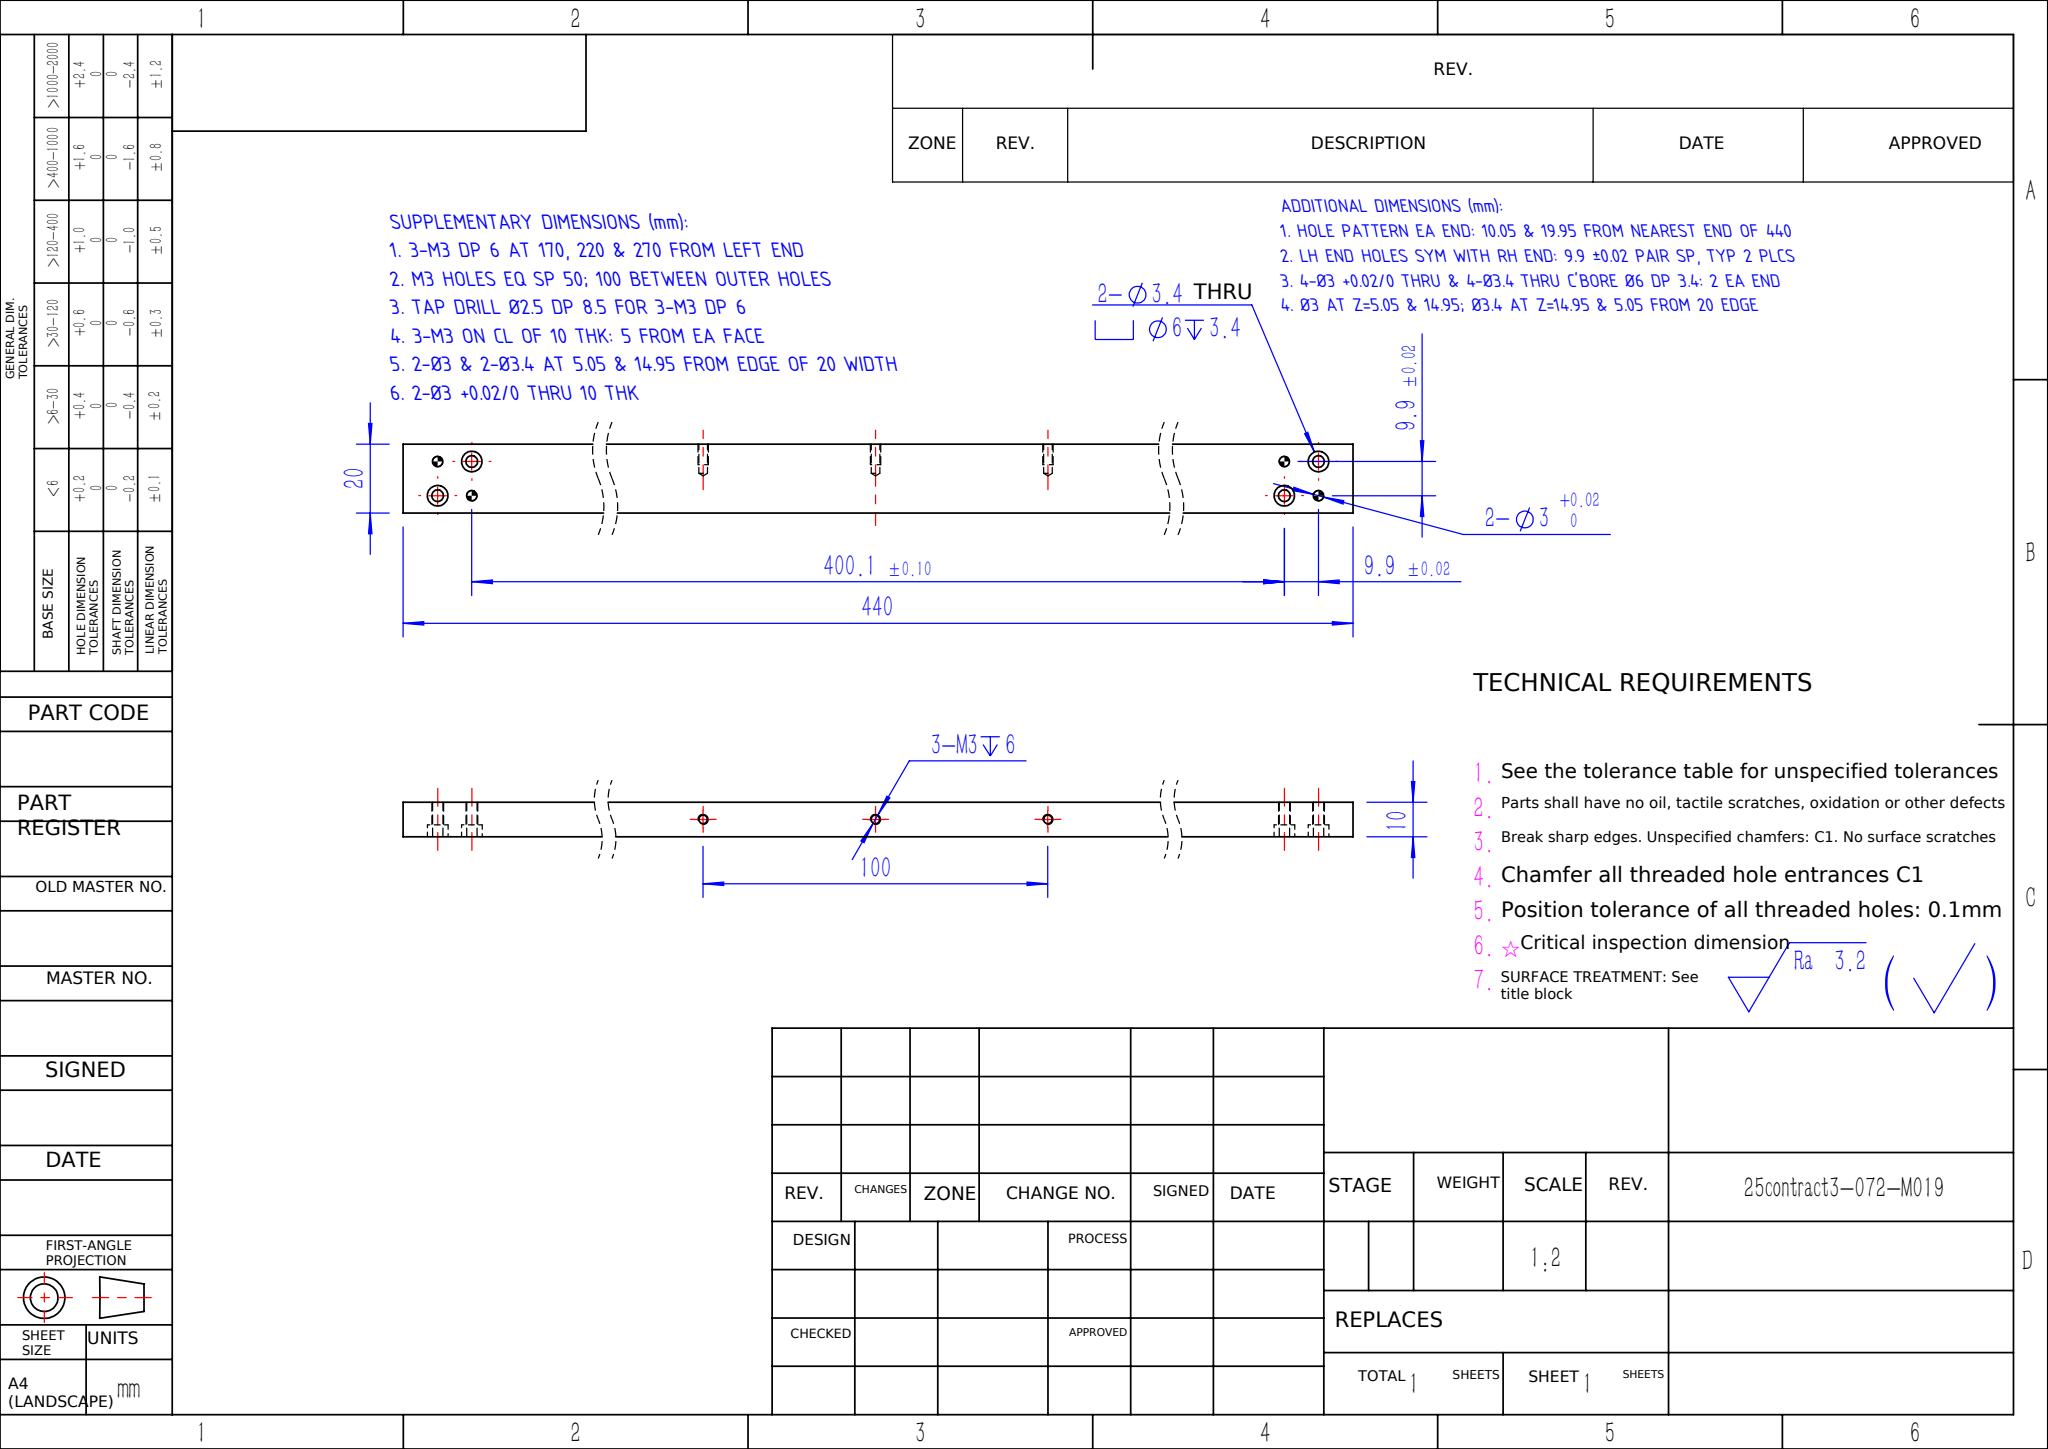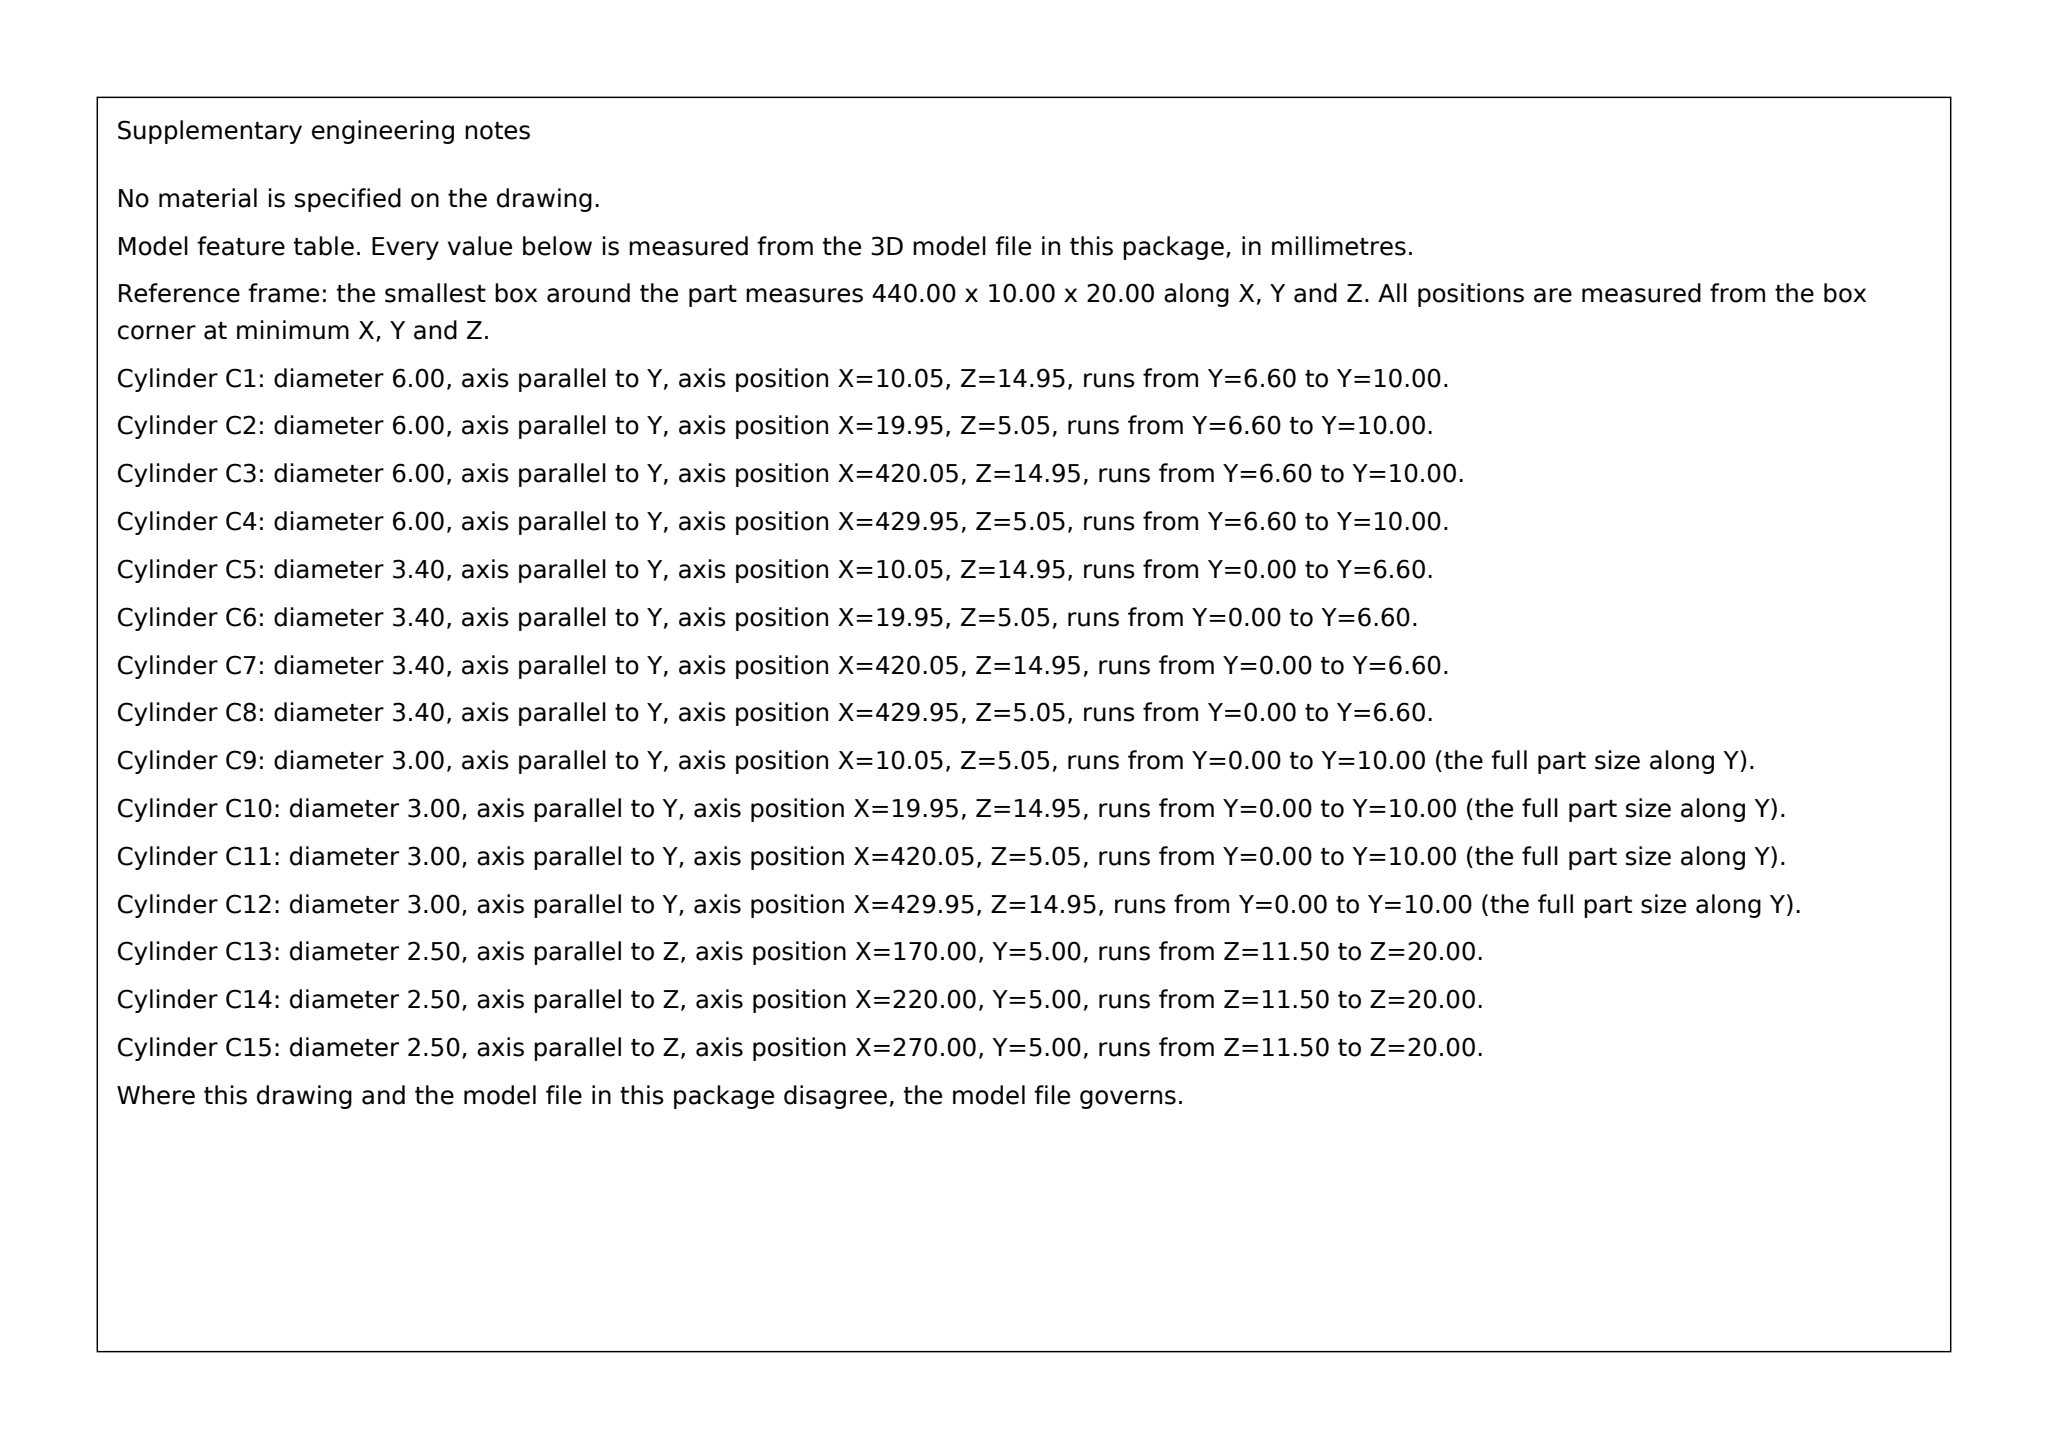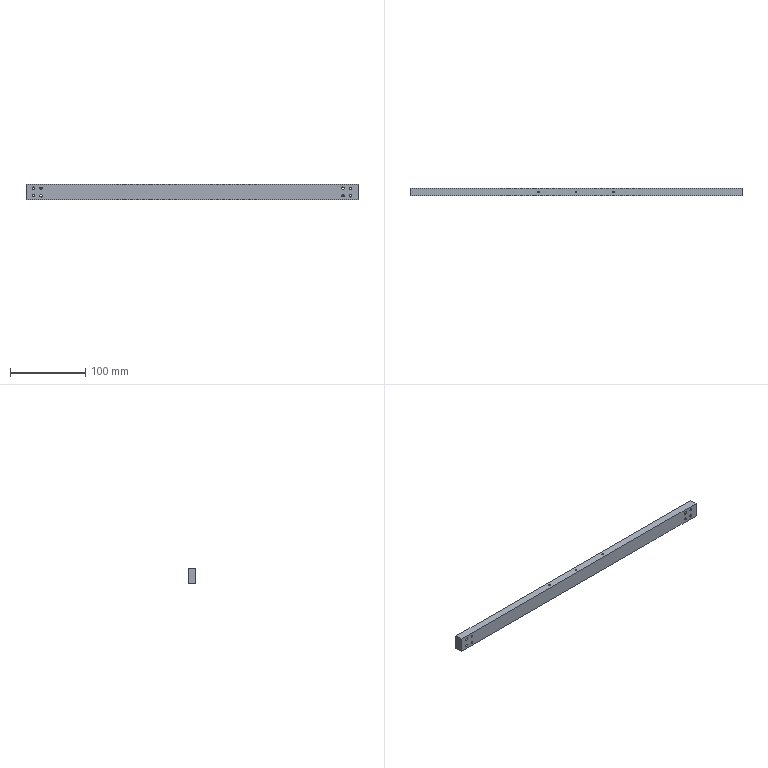Part | SolidWorks | mm | 1 solid | 46 faces | box 440 x 10 x 20 mm | volume 86964 mm3 | cylinder 30 | plane 10 | cone 6 | commonest cylinder face diameters 3 x8 6 x8 3.4 x8 2.5 x6
build123d program:
from build123d import *

# Parameters (mm, degrees)
SKETCH7_W                                         = 440
SKETCH7_H                                         = 20
BOSS_EXTRUDE1_DEPTH                               = 10
HOLE_SIZE_ACCORDING_TO_HEXAGON_SOCKET_D           = 3.4
HOLE_SIZE_ACCORDING_TO_HEXAGON_SOCKET_CBORE_D     = 6
HOLE_SIZE_ACCORDING_TO_HEXAGON_SOCKET_CBORE_DEPTH = 3.4
SIZE_MM_DOWEL_PIN_HOLE1_D                         = 3
M3_TAPPED_HOLE1_D                                 = 2.5
M3_TAPPED_HOLE1_DEPTH                             = 8.5
M3_TAPPED_HOLE1_TIP                               = 0.7511
HOLE_SIZE_ACCORDING_TO_HEXAGON_SO_2_D             = 3.4
HOLE_SIZE_ACCORDING_TO_HEXAGON_SO_2_CBORE_D       = 6
HOLE_SIZE_ACCORDING_TO_HEXAGON_SO_2_CBORE_DEPTH   = 3.4
SIZE_MM_DOWEL_PIN_HOLE2_D                         = 3


with BuildPart() as part:
    # Sketch7 → Boss-Extrude1 (new body)
    with BuildSketch(Plane(origin=(0, 0, 0), x_dir=(1, 0, 0), z_dir=(0, 1, 0))):
        Rectangle(SKETCH7_W, SKETCH7_H)
    extrude(amount=BOSS_EXTRUDE1_DEPTH)

    # Hole Size _ according to_ Hexagon Socket (through all)
    with Locations(Plane(origin=(0, 10, 0), x_dir=(1, 0, 0), z_dir=(0, 1, 0))):
        with Locations((-200.05, 4.95), (-209.95, -4.95)):
            CounterBoreHole(HOLE_SIZE_ACCORDING_TO_HEXAGON_SOCKET_D / 2, HOLE_SIZE_ACCORDING_TO_HEXAGON_SOCKET_CBORE_D / 2, HOLE_SIZE_ACCORDING_TO_HEXAGON_SOCKET_CBORE_DEPTH)

    # Size mm Dowel Pin Hole1 (through all)
    with Locations(Plane(origin=(0, 10, 0), x_dir=(1, 0, 0), z_dir=(0, 1, 0))):
        with Locations((-209.95, 4.95), (-200.05, -4.95)):
            Hole(SIZE_MM_DOWEL_PIN_HOLE1_D / 2)

    # M3 Tapped Hole1
    with Locations(Plane.XY.offset(10)):
        with Locations((0, 5), (50, 5), (-50, 5)):
            Hole(M3_TAPPED_HOLE1_D / 2, depth=M3_TAPPED_HOLE1_DEPTH)
            with Locations((0, 0, -(M3_TAPPED_HOLE1_DEPTH + M3_TAPPED_HOLE1_TIP / 2))):  # 118° drill point
                Cone(0, M3_TAPPED_HOLE1_D / 2, M3_TAPPED_HOLE1_TIP, mode=Mode.SUBTRACT)

    # Hole Size _ according to_ Hexagon So 2 (through all)
    with Locations(Plane(origin=(0, 10, 0), x_dir=(1, 0, 0), z_dir=(0, 1, 0))):
        with Locations((209.95, 4.95), (200.05, -4.95)):
            CounterBoreHole(HOLE_SIZE_ACCORDING_TO_HEXAGON_SO_2_D / 2, HOLE_SIZE_ACCORDING_TO_HEXAGON_SO_2_CBORE_D / 2, HOLE_SIZE_ACCORDING_TO_HEXAGON_SO_2_CBORE_DEPTH)

    # Size mm Dowel Pin Hole2 (through all)
    with Locations(Plane(origin=(0, 10, 0), x_dir=(1, 0, 0), z_dir=(0, 1, 0))):
        with Locations((200.05, 4.95), (209.95, -4.95)):
            Hole(SIZE_MM_DOWEL_PIN_HOLE2_D / 2)


solid = part.part